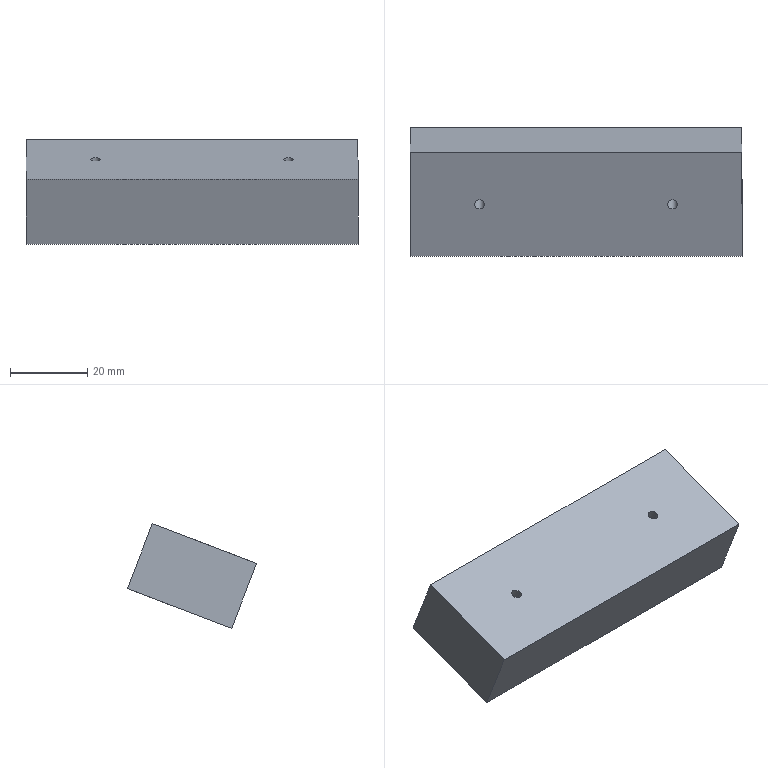Component | SolidWorks | CV-BA-74X27-1 | 1 solid | 19 faces | box 86 x 33.42 x 27.14 mm | volume 43255 mm3 | plane 11 | cylinder 4 | cone 4 | commonest cylinder face diameters 2.5 x4
build123d program:
from build123d import *

# Parameters (mm, degrees)
SKETCH1_W             = 86
SKETCH1_H             = 28.9
BOSS_EXTRUDE1_DEPTH   = 18
SKETCH2_W             = 57.364
SKETCH2_H             = 24.341
CUT_EXTRUDE1_DEPTH    = 1
M3_TAPPED_HOLE1_D     = 2.5
M3_TAPPED_HOLE1_DEPTH = 8.5
M3_TAPPED_HOLE1_TIP   = 0.7511


with BuildPart() as part:
    # Sketch1 → Boss-Extrude1 (new body)
    with BuildSketch(Plane.XY):
        Rectangle(SKETCH1_W, SKETCH1_H)
    extrude(amount=BOSS_EXTRUDE1_DEPTH)

    # Sketch2 → Cut-Extrude1 (cut)
    with BuildSketch(Plane.XY.offset(18)):
        Rectangle(SKETCH2_W, SKETCH2_H)
    extrude(amount=-CUT_EXTRUDE1_DEPTH, mode=Mode.SUBTRACT)

    # M3 Tapped Hole1
    with Locations(Plane(origin=(0, 0, 0), x_dir=(-1, 0, 0), z_dir=(0, 0, -1))):
        with Locations((-25, 0), (25, 0)):
            Hole(M3_TAPPED_HOLE1_D / 2, depth=M3_TAPPED_HOLE1_DEPTH)
            with Locations((0, 0, -(M3_TAPPED_HOLE1_DEPTH + M3_TAPPED_HOLE1_TIP / 2))):  # 118° drill point
                Cone(0, M3_TAPPED_HOLE1_D / 2, M3_TAPPED_HOLE1_TIP, mode=Mode.SUBTRACT)


solid = part.part

# Placed as in the assembly
solid = solid.moved(Location((-143.297, 122.354, 409.108), (-159.065, 0, 0)))
STEP:
#1=COLOUR_RGB('',0.7922,0.8196,0.9333);
#2=FILL_AREA_STYLE_COLOUR('',#1);
#3=FILL_AREA_STYLE('',(#2));
#4=SURFACE_STYLE_FILL_AREA(#3);
#5=SURFACE_SIDE_STYLE('',(#4));
#6=SURFACE_STYLE_USAGE(.BOTH.,#5);
#7=PRESENTATION_STYLE_ASSIGNMENT((#6));
#8=CARTESIAN_POINT('',(-4.608,4.937,15.794));
#9=VERTEX_POINT('',#8);
#10=CARTESIAN_POINT('',(-4.707,4.937,15.794));
#11=VERTEX_POINT('',#10);
#12=CARTESIAN_POINT('',(-4.657,4.937,15.794));
#13=DIRECTION('',(0.,-0.3573,0.934));
#14=DIRECTION('',(-1.,0.,0.));
#15=AXIS2_PLACEMENT_3D('',#12,#13,#14);
#16=CIRCLE('',#15,0.04921);
#17=EDGE_CURVE('',#9,#11,#16,.T.);
#18=ORIENTED_EDGE('',*,*,#17,.F.);
#19=CARTESIAN_POINT('',(-4.608,4.817,16.107));
#20=VERTEX_POINT('',#19);
#21=CARTESIAN_POINT('',(-4.608,4.817,16.107));
#22=DIRECTION('',(0.,-0.3573,0.934));
#23=VECTOR('',#22,39.37);
#24=LINE('',#21,#23);
#25=EDGE_CURVE('',#9,#20,#24,.T.);
#26=ORIENTED_EDGE('',*,*,#25,.T.);
#27=CARTESIAN_POINT('',(-4.707,4.817,16.107));
#28=VERTEX_POINT('',#27);
#29=CARTESIAN_POINT('',(-4.657,4.817,16.107));
#30=DIRECTION('',(0.,-0.3573,0.934));
#31=DIRECTION('',(-1.,0.,0.));
#32=AXIS2_PLACEMENT_3D('',#29,#30,#31);
#33=CIRCLE('',#32,0.04921);
#34=EDGE_CURVE('',#20,#28,#33,.T.);
#35=ORIENTED_EDGE('',*,*,#34,.T.);
#36=CARTESIAN_POINT('',(-4.707,4.817,16.107));
#37=DIRECTION('',(0.,-0.3573,0.934));
#38=VECTOR('',#37,39.37);
#39=LINE('',#36,#38);
#40=EDGE_CURVE('',#11,#28,#39,.T.);
#41=ORIENTED_EDGE('',*,*,#40,.F.);
#42=EDGE_LOOP('',(#18,#26,#35,#41));
#43=FACE_OUTER_BOUND('',#42,.T.);
#44=CARTESIAN_POINT('',(-4.657,4.817,16.107));
#45=DIRECTION('',(0.,-0.3573,0.934));
#46=DIRECTION('',(-1.,0.,0.));
#47=AXIS2_PLACEMENT_3D('',#44,#45,#46);
#48=CYLINDRICAL_SURFACE('',#47,0.04921);
#49=ADVANCED_FACE('',(#43),#48,.F.);
#50=CARTESIAN_POINT('',(-4.657,4.947,15.766));
#51=VERTEX_POINT('',#50);
#52=CARTESIAN_POINT('',(-4.707,4.937,15.794));
#53=DIRECTION('',(-0.8572,-0.184,0.481));
#54=VECTOR('',#53,39.37);
#55=LINE('',#52,#54);
#56=EDGE_CURVE('',#51,#11,#55,.T.);
#57=ORIENTED_EDGE('',*,*,#56,.F.);
#58=CARTESIAN_POINT('',(-4.608,4.937,15.794));
#59=DIRECTION('',(0.8572,-0.184,0.481));
#60=VECTOR('',#59,39.37);
#61=LINE('',#58,#60);
#62=EDGE_CURVE('',#51,#9,#61,.T.);
#63=ORIENTED_EDGE('',*,*,#62,.T.);
#64=ORIENTED_EDGE('',*,*,#17,.T.);
#65=EDGE_LOOP('',(#57,#63,#64));
#66=FACE_OUTER_BOUND('',#65,.T.);
#67=CARTESIAN_POINT('',(-4.657,4.937,15.794));
#68=DIRECTION('',(0.,-0.3573,0.934));
#69=DIRECTION('',(-1.,0.,0.));
#70=AXIS2_PLACEMENT_3D('',#67,#68,#69);
#71=CONICAL_SURFACE('',#70,0.04921,1.03);
#72=ADVANCED_FACE('',(#66),#71,.F.);
#73=CARTESIAN_POINT('',(-6.577,4.937,15.794));
#74=VERTEX_POINT('',#73);
#75=CARTESIAN_POINT('',(-6.675,4.937,15.794));
#76=VERTEX_POINT('',#75);
#77=CARTESIAN_POINT('',(-6.626,4.937,15.794));
#78=DIRECTION('',(0.,-0.3573,0.934));
#79=DIRECTION('',(-1.,0.,0.));
#80=AXIS2_PLACEMENT_3D('',#77,#78,#79);
#81=CIRCLE('',#80,0.04921);
#82=EDGE_CURVE('',#74,#76,#81,.T.);
#83=ORIENTED_EDGE('',*,*,#82,.F.);
#84=CARTESIAN_POINT('',(-6.577,4.817,16.107));
#85=VERTEX_POINT('',#84);
#86=CARTESIAN_POINT('',(-6.577,4.817,16.107));
#87=DIRECTION('',(0.,-0.3573,0.934));
#88=VECTOR('',#87,39.37);
#89=LINE('',#86,#88);
#90=EDGE_CURVE('',#74,#85,#89,.T.);
#91=ORIENTED_EDGE('',*,*,#90,.T.);
#92=CARTESIAN_POINT('',(-6.675,4.817,16.107));
#93=VERTEX_POINT('',#92);
#94=CARTESIAN_POINT('',(-6.626,4.817,16.107));
#95=DIRECTION('',(0.,-0.3573,0.934));
#96=DIRECTION('',(-1.,0.,0.));
#97=AXIS2_PLACEMENT_3D('',#94,#95,#96);
#98=CIRCLE('',#97,0.04921);
#99=EDGE_CURVE('',#85,#93,#98,.T.);
#100=ORIENTED_EDGE('',*,*,#99,.T.);
#101=CARTESIAN_POINT('',(-6.675,4.817,16.107));
#102=DIRECTION('',(0.,-0.3573,0.934));
#103=VECTOR('',#102,39.37);
#104=LINE('',#101,#103);
#105=EDGE_CURVE('',#76,#93,#104,.T.);
#106=ORIENTED_EDGE('',*,*,#105,.F.);
#107=EDGE_LOOP('',(#83,#91,#100,#106));
#108=FACE_OUTER_BOUND('',#107,.T.);
#109=CARTESIAN_POINT('',(-6.626,4.817,16.107));
#110=DIRECTION('',(0.,-0.3573,0.934));
#111=DIRECTION('',(-1.,0.,0.));
#112=AXIS2_PLACEMENT_3D('',#109,#110,#111);
#113=CYLINDRICAL_SURFACE('',#112,0.04921);
#114=ADVANCED_FACE('',(#108),#113,.F.);
#115=CARTESIAN_POINT('',(-6.626,4.947,15.766));
#116=VERTEX_POINT('',#115);
#117=CARTESIAN_POINT('',(-6.675,4.937,15.794));
#118=DIRECTION('',(-0.8572,-0.184,0.481));
#119=VECTOR('',#118,39.37);
#120=LINE('',#117,#119);
#121=EDGE_CURVE('',#116,#76,#120,.T.);
#122=ORIENTED_EDGE('',*,*,#121,.F.);
#123=CARTESIAN_POINT('',(-6.577,4.937,15.794));
#124=DIRECTION('',(0.8572,-0.184,0.481));
#125=VECTOR('',#124,39.37);
#126=LINE('',#123,#125);
#127=EDGE_CURVE('',#116,#74,#126,.T.);
#128=ORIENTED_EDGE('',*,*,#127,.T.);
#129=ORIENTED_EDGE('',*,*,#82,.T.);
#130=EDGE_LOOP('',(#122,#128,#129));
#131=FACE_OUTER_BOUND('',#130,.T.);
#132=CARTESIAN_POINT('',(-6.626,4.937,15.794));
#133=DIRECTION('',(0.,-0.3573,0.934));
#134=DIRECTION('',(-1.,0.,0.));
#135=AXIS2_PLACEMENT_3D('',#132,#133,#134);
#136=CONICAL_SURFACE('',#135,0.04921,1.03);
#137=ADVANCED_FACE('',(#131),#136,.F.);
#138=CARTESIAN_POINT('',(-3.949,5.348,16.31));
#139=VERTEX_POINT('',#138);
#140=CARTESIAN_POINT('',(-3.949,4.286,15.903));
#141=VERTEX_POINT('',#140);
#142=CARTESIAN_POINT('',(-3.949,4.286,15.903));
#143=DIRECTION('',(0.,-0.934,-0.3573));
#144=VECTOR('',#143,39.37);
#145=LINE('',#142,#144);
#146=EDGE_CURVE('',#139,#141,#145,.T.);
#147=ORIENTED_EDGE('',*,*,#146,.T.);
#148=CARTESIAN_POINT('',(-3.949,4.539,15.241));
#149=VERTEX_POINT('',#148);
#150=CARTESIAN_POINT('',(-3.949,4.539,15.241));
#151=DIRECTION('',(0.,-0.3573,0.934));
#152=VECTOR('',#151,39.37);
#153=LINE('',#150,#152);
#154=EDGE_CURVE('',#149,#141,#153,.T.);
#155=ORIENTED_EDGE('',*,*,#154,.F.);
#156=CARTESIAN_POINT('',(-3.949,5.602,15.648));
#157=VERTEX_POINT('',#156);
#158=CARTESIAN_POINT('',(-3.949,4.539,15.241));
#159=DIRECTION('',(0.,-0.934,-0.3573));
#160=VECTOR('',#159,39.37);
#161=LINE('',#158,#160);
#162=EDGE_CURVE('',#157,#149,#161,.T.);
#163=ORIENTED_EDGE('',*,*,#162,.F.);
#164=CARTESIAN_POINT('',(-3.949,5.602,15.648));
#165=DIRECTION('',(0.,-0.3573,0.934));
#166=VECTOR('',#165,39.37);
#167=LINE('',#164,#166);
#168=EDGE_CURVE('',#157,#139,#167,.T.);
#169=ORIENTED_EDGE('',*,*,#168,.T.);
#170=EDGE_LOOP('',(#147,#155,#163,#169));
#171=FACE_OUTER_BOUND('',#170,.T.);
#172=CARTESIAN_POINT('',(-3.949,4.539,15.241));
#173=DIRECTION('',(-1.,-0.,0.));
#174=DIRECTION('',(-0.,0.3573,-0.934));
#175=AXIS2_PLACEMENT_3D('',#172,#173,#174);
#176=PLANE('',#175);
#177=ADVANCED_FACE('',(#171),#176,.F.);
#178=CARTESIAN_POINT('',(-7.335,4.286,15.903));
#179=VERTEX_POINT('',#178);
#180=CARTESIAN_POINT('',(-7.335,4.286,15.903));
#181=DIRECTION('',(-1.,-0.,0.));
#182=VECTOR('',#181,39.37);
#183=LINE('',#180,#182);
#184=EDGE_CURVE('',#141,#179,#183,.T.);
#185=ORIENTED_EDGE('',*,*,#184,.T.);
#186=CARTESIAN_POINT('',(-7.335,4.539,15.241));
#187=VERTEX_POINT('',#186);
#188=CARTESIAN_POINT('',(-7.335,4.539,15.241));
#189=DIRECTION('',(0.,-0.3573,0.934));
#190=VECTOR('',#189,39.37);
#191=LINE('',#188,#190);
#192=EDGE_CURVE('',#187,#179,#191,.T.);
#193=ORIENTED_EDGE('',*,*,#192,.F.);
#194=CARTESIAN_POINT('',(-7.335,4.539,15.241));
#195=DIRECTION('',(-1.,-0.,0.));
#196=VECTOR('',#195,39.37);
#197=LINE('',#194,#196);
#198=EDGE_CURVE('',#149,#187,#197,.T.);
#199=ORIENTED_EDGE('',*,*,#198,.F.);
#200=ORIENTED_EDGE('',*,*,#154,.T.);
#201=EDGE_LOOP('',(#185,#193,#199,#200));
#202=FACE_OUTER_BOUND('',#201,.T.);
#203=CARTESIAN_POINT('',(-7.335,4.539,15.241));
#204=DIRECTION('',(-0.,0.934,0.3573));
#205=DIRECTION('',(0.,-0.3573,0.934));
#206=AXIS2_PLACEMENT_3D('',#203,#204,#205);
#207=PLANE('',#206);
#208=ADVANCED_FACE('',(#202),#207,.F.);
#209=CARTESIAN_POINT('',(-7.335,5.348,16.31));
#210=VERTEX_POINT('',#209);
#211=CARTESIAN_POINT('',(-7.335,4.286,15.903));
#212=DIRECTION('',(0.,0.934,0.3573));
#213=VECTOR('',#212,39.37);
#214=LINE('',#211,#213);
#215=EDGE_CURVE('',#179,#210,#214,.T.);
#216=ORIENTED_EDGE('',*,*,#215,.T.);
#217=CARTESIAN_POINT('',(-7.335,5.602,15.648));
#218=VERTEX_POINT('',#217);
#219=CARTESIAN_POINT('',(-7.335,5.602,15.648));
#220=DIRECTION('',(0.,-0.3573,0.934));
#221=VECTOR('',#220,39.37);
#222=LINE('',#219,#221);
#223=EDGE_CURVE('',#218,#210,#222,.T.);
#224=ORIENTED_EDGE('',*,*,#223,.F.);
#225=CARTESIAN_POINT('',(-7.335,4.539,15.241));
#226=DIRECTION('',(0.,0.934,0.3573));
#227=VECTOR('',#226,39.37);
#228=LINE('',#225,#227);
#229=EDGE_CURVE('',#187,#218,#228,.T.);
#230=ORIENTED_EDGE('',*,*,#229,.F.);
#231=ORIENTED_EDGE('',*,*,#192,.T.);
#232=EDGE_LOOP('',(#216,#224,#230,#231));
#233=FACE_OUTER_BOUND('',#232,.T.);
#234=CARTESIAN_POINT('',(-7.335,4.539,15.241));
#235=DIRECTION('',(1.,-0.,-0.));
#236=DIRECTION('',(-0.,-0.934,-0.3573));
#237=AXIS2_PLACEMENT_3D('',#234,#235,#236);
#238=PLANE('',#237);
#239=ADVANCED_FACE('',(#233),#238,.F.);
#240=CARTESIAN_POINT('',(-7.335,5.348,16.31));
#241=DIRECTION('',(1.,0.,-0.));
#242=VECTOR('',#241,39.37);
#243=LINE('',#240,#242);
#244=EDGE_CURVE('',#210,#139,#243,.T.);
#245=ORIENTED_EDGE('',*,*,#244,.T.);
#246=ORIENTED_EDGE('',*,*,#168,.F.);
#247=CARTESIAN_POINT('',(-7.335,5.602,15.648));
#248=DIRECTION('',(1.,0.,-0.));
#249=VECTOR('',#248,39.37);
#250=LINE('',#247,#249);
#251=EDGE_CURVE('',#218,#157,#250,.T.);
#252=ORIENTED_EDGE('',*,*,#251,.F.);
#253=ORIENTED_EDGE('',*,*,#223,.T.);
#254=EDGE_LOOP('',(#245,#246,#252,#253));
#255=FACE_OUTER_BOUND('',#254,.T.);
#256=CARTESIAN_POINT('',(-7.335,5.602,15.648));
#257=DIRECTION('',(0.,-0.934,-0.3573));
#258=DIRECTION('',(-0.,0.3573,-0.934));
#259=AXIS2_PLACEMENT_3D('',#256,#257,#258);
#260=PLANE('',#259);
#261=ADVANCED_FACE('',(#255),#260,.F.);
#262=CARTESIAN_POINT('',(-4.512,5.518,15.616));
#263=VERTEX_POINT('',#262);
#264=CARTESIAN_POINT('',(-4.512,4.623,15.274));
#265=VERTEX_POINT('',#264);
#266=CARTESIAN_POINT('',(-4.512,4.623,15.274));
#267=DIRECTION('',(0.,-0.934,-0.3573));
#268=VECTOR('',#267,39.37);
#269=LINE('',#266,#268);
#270=EDGE_CURVE('',#263,#265,#269,.T.);
#271=ORIENTED_EDGE('',*,*,#270,.F.);
#272=CARTESIAN_POINT('',(-6.771,5.518,15.616));
#273=VERTEX_POINT('',#272);
#274=CARTESIAN_POINT('',(-6.771,5.518,15.616));
#275=DIRECTION('',(1.,0.,0.));
#276=VECTOR('',#275,39.37);
#277=LINE('',#274,#276);
#278=EDGE_CURVE('',#273,#263,#277,.T.);
#279=ORIENTED_EDGE('',*,*,#278,.F.);
#280=CARTESIAN_POINT('',(-6.771,4.623,15.274));
#281=VERTEX_POINT('',#280);
#282=CARTESIAN_POINT('',(-6.771,4.623,15.274));
#283=DIRECTION('',(0.,0.934,0.3573));
#284=VECTOR('',#283,39.37);
#285=LINE('',#282,#284);
#286=EDGE_CURVE('',#281,#273,#285,.T.);
#287=ORIENTED_EDGE('',*,*,#286,.F.);
#288=CARTESIAN_POINT('',(-6.771,4.623,15.274));
#289=DIRECTION('',(-1.,-0.,0.));
#290=VECTOR('',#289,39.37);
#291=LINE('',#288,#290);
#292=EDGE_CURVE('',#265,#281,#291,.T.);
#293=ORIENTED_EDGE('',*,*,#292,.F.);
#294=EDGE_LOOP('',(#271,#279,#287,#293));
#295=FACE_BOUND('',#294,.T.);
#296=ORIENTED_EDGE('',*,*,#162,.T.);
#297=ORIENTED_EDGE('',*,*,#198,.T.);
#298=ORIENTED_EDGE('',*,*,#229,.T.);
#299=ORIENTED_EDGE('',*,*,#251,.T.);
#300=EDGE_LOOP('',(#296,#297,#298,#299));
#301=FACE_OUTER_BOUND('',#300,.T.);
#302=CARTESIAN_POINT('',(-5.642,5.07,15.445));
#303=DIRECTION('',(-0.,0.3573,-0.934));
#304=DIRECTION('',(1.,0.,-0.));
#305=AXIS2_PLACEMENT_3D('',#302,#303,#304);
#306=PLANE('',#305);
#307=ADVANCED_FACE('',(#295,#301),#306,.T.);
#308=CARTESIAN_POINT('',(-4.657,4.817,16.107));
#309=DIRECTION('',(0.,-0.3573,0.934));
#310=DIRECTION('',(-1.,0.,0.));
#311=AXIS2_PLACEMENT_3D('',#308,#309,#310);
#312=CIRCLE('',#311,0.04921);
#313=EDGE_CURVE('',#28,#20,#312,.T.);
#314=ORIENTED_EDGE('',*,*,#313,.F.);
#315=ORIENTED_EDGE('',*,*,#34,.F.);
#316=EDGE_LOOP('',(#314,#315));
#317=FACE_BOUND('',#316,.T.);
#318=CARTESIAN_POINT('',(-6.626,4.817,16.107));
#319=DIRECTION('',(0.,-0.3573,0.934));
#320=DIRECTION('',(-1.,0.,0.));
#321=AXIS2_PLACEMENT_3D('',#318,#319,#320);
#322=CIRCLE('',#321,0.04921);
#323=EDGE_CURVE('',#93,#85,#322,.T.);
#324=ORIENTED_EDGE('',*,*,#323,.F.);
#325=ORIENTED_EDGE('',*,*,#99,.F.);
#326=EDGE_LOOP('',(#324,#325));
#327=FACE_BOUND('',#326,.T.);
#328=ORIENTED_EDGE('',*,*,#146,.F.);
#329=ORIENTED_EDGE('',*,*,#244,.F.);
#330=ORIENTED_EDGE('',*,*,#215,.F.);
#331=ORIENTED_EDGE('',*,*,#184,.F.);
#332=EDGE_LOOP('',(#328,#329,#330,#331));
#333=FACE_OUTER_BOUND('',#332,.T.);
#334=CARTESIAN_POINT('',(-5.642,4.817,16.107));
#335=DIRECTION('',(-0.,0.3573,-0.934));
#336=DIRECTION('',(1.,0.,-0.));
#337=AXIS2_PLACEMENT_3D('',#334,#335,#336);
#338=PLANE('',#337);
#339=ADVANCED_FACE('',(#317,#327,#333),#338,.F.);
#340=ORIENTED_EDGE('',*,*,#270,.T.);
#341=CARTESIAN_POINT('',(-4.512,4.609,15.31));
#342=VERTEX_POINT('',#341);
#343=CARTESIAN_POINT('',(-4.512,4.609,15.31));
#344=DIRECTION('',(-0.,0.3573,-0.934));
#345=VECTOR('',#344,39.37);
#346=LINE('',#343,#345);
#347=EDGE_CURVE('',#342,#265,#346,.T.);
#348=ORIENTED_EDGE('',*,*,#347,.F.);
#349=CARTESIAN_POINT('',(-4.512,5.504,15.653));
#350=VERTEX_POINT('',#349);
#351=CARTESIAN_POINT('',(-4.512,4.609,15.31));
#352=DIRECTION('',(0.,-0.934,-0.3573));
#353=VECTOR('',#352,39.37);
#354=LINE('',#351,#353);
#355=EDGE_CURVE('',#350,#342,#354,.T.);
#356=ORIENTED_EDGE('',*,*,#355,.F.);
#357=CARTESIAN_POINT('',(-4.512,5.504,15.653));
#358=DIRECTION('',(-0.,0.3573,-0.934));
#359=VECTOR('',#358,39.37);
#360=LINE('',#357,#359);
#361=EDGE_CURVE('',#350,#263,#360,.T.);
#362=ORIENTED_EDGE('',*,*,#361,.T.);
#363=EDGE_LOOP('',(#340,#348,#356,#362));
#364=FACE_OUTER_BOUND('',#363,.T.);
#365=CARTESIAN_POINT('',(-4.512,4.609,15.31));
#366=DIRECTION('',(1.,0.,-0.));
#367=DIRECTION('',(0.,-0.3573,0.934));
#368=AXIS2_PLACEMENT_3D('',#365,#366,#367);
#369=PLANE('',#368);
#370=ADVANCED_FACE('',(#364),#369,.F.);
#371=ORIENTED_EDGE('',*,*,#278,.T.);
#372=ORIENTED_EDGE('',*,*,#361,.F.);
#373=CARTESIAN_POINT('',(-6.771,5.504,15.653));
#374=VERTEX_POINT('',#373);
#375=CARTESIAN_POINT('',(-6.771,5.504,15.653));
#376=DIRECTION('',(1.,0.,0.));
#377=VECTOR('',#376,39.37);
#378=LINE('',#375,#377);
#379=EDGE_CURVE('',#374,#350,#378,.T.);
#380=ORIENTED_EDGE('',*,*,#379,.F.);
#381=CARTESIAN_POINT('',(-6.771,5.504,15.653));
#382=DIRECTION('',(-0.,0.3573,-0.934));
#383=VECTOR('',#382,39.37);
#384=LINE('',#381,#383);
#385=EDGE_CURVE('',#374,#273,#384,.T.);
#386=ORIENTED_EDGE('',*,*,#385,.T.);
#387=EDGE_LOOP('',(#371,#372,#380,#386));
#388=FACE_OUTER_BOUND('',#387,.T.);
#389=CARTESIAN_POINT('',(-6.771,5.504,15.653));
#390=DIRECTION('',(-0.,0.934,0.3573));
#391=DIRECTION('',(1.,0.,0.));
#392=AXIS2_PLACEMENT_3D('',#389,#390,#391);
#393=PLANE('',#392);
#394=ADVANCED_FACE('',(#388),#393,.F.);
#395=ORIENTED_EDGE('',*,*,#286,.T.);
#396=ORIENTED_EDGE('',*,*,#385,.F.);
#397=CARTESIAN_POINT('',(-6.771,4.609,15.31));
#398=VERTEX_POINT('',#397);
#399=CARTESIAN_POINT('',(-6.771,4.609,15.31));
#400=DIRECTION('',(0.,0.934,0.3573));
#401=VECTOR('',#400,39.37);
#402=LINE('',#399,#401);
#403=EDGE_CURVE('',#398,#374,#402,.T.);
#404=ORIENTED_EDGE('',*,*,#403,.F.);
#405=CARTESIAN_POINT('',(-6.771,4.609,15.31));
#406=DIRECTION('',(-0.,0.3573,-0.934));
#407=VECTOR('',#406,39.37);
#408=LINE('',#405,#407);
#409=EDGE_CURVE('',#398,#281,#408,.T.);
#410=ORIENTED_EDGE('',*,*,#409,.T.);
#411=EDGE_LOOP('',(#395,#396,#404,#410));
#412=FACE_OUTER_BOUND('',#411,.T.);
#413=CARTESIAN_POINT('',(-6.771,4.609,15.31));
#414=DIRECTION('',(-1.,-0.,0.));
#415=DIRECTION('',(0.,0.934,0.3573));
#416=AXIS2_PLACEMENT_3D('',#413,#414,#415);
#417=PLANE('',#416);
#418=ADVANCED_FACE('',(#412),#417,.F.);
#419=ORIENTED_EDGE('',*,*,#292,.T.);
#420=ORIENTED_EDGE('',*,*,#409,.F.);
#421=CARTESIAN_POINT('',(-6.771,4.609,15.31));
#422=DIRECTION('',(-1.,-0.,0.));
#423=VECTOR('',#422,39.37);
#424=LINE('',#421,#423);
#425=EDGE_CURVE('',#342,#398,#424,.T.);
#426=ORIENTED_EDGE('',*,*,#425,.F.);
#427=ORIENTED_EDGE('',*,*,#347,.T.);
#428=EDGE_LOOP('',(#419,#420,#426,#427));
#429=FACE_OUTER_BOUND('',#428,.T.);
#430=CARTESIAN_POINT('',(-6.771,4.609,15.31));
#431=DIRECTION('',(0.,-0.934,-0.3573));
#432=DIRECTION('',(-0.,0.3573,-0.934));
#433=AXIS2_PLACEMENT_3D('',#430,#431,#432);
#434=PLANE('',#433);
#435=ADVANCED_FACE('',(#429),#434,.F.);
#436=ORIENTED_EDGE('',*,*,#355,.T.);
#437=ORIENTED_EDGE('',*,*,#425,.T.);
#438=ORIENTED_EDGE('',*,*,#403,.T.);
#439=ORIENTED_EDGE('',*,*,#379,.T.);
#440=EDGE_LOOP('',(#436,#437,#438,#439));
#441=FACE_OUTER_BOUND('',#440,.T.);
#442=CARTESIAN_POINT('',(-5.642,5.056,15.482));
#443=DIRECTION('',(-0.,0.3573,-0.934));
#444=DIRECTION('',(1.,0.,-0.));
#445=AXIS2_PLACEMENT_3D('',#442,#443,#444);
#446=PLANE('',#445);
#447=ADVANCED_FACE('',(#441),#446,.T.);
#448=ORIENTED_EDGE('',*,*,#127,.F.);
#449=ORIENTED_EDGE('',*,*,#121,.T.);
#450=CARTESIAN_POINT('',(-6.626,4.937,15.794));
#451=DIRECTION('',(0.,-0.3573,0.934));
#452=DIRECTION('',(-1.,0.,0.));
#453=AXIS2_PLACEMENT_3D('',#450,#451,#452);
#454=CIRCLE('',#453,0.04921);
#455=EDGE_CURVE('',#76,#74,#454,.T.);
#456=ORIENTED_EDGE('',*,*,#455,.T.);
#457=EDGE_LOOP('',(#448,#449,#456));
#458=FACE_OUTER_BOUND('',#457,.T.);
#459=CARTESIAN_POINT('',(-6.626,4.937,15.794));
#460=DIRECTION('',(0.,-0.3573,0.934));
#461=DIRECTION('',(-1.,0.,0.));
#462=AXIS2_PLACEMENT_3D('',#459,#460,#461);
#463=CONICAL_SURFACE('',#462,0.04921,1.03);
#464=ADVANCED_FACE('',(#458),#463,.F.);
#465=ORIENTED_EDGE('',*,*,#90,.F.);
#466=ORIENTED_EDGE('',*,*,#455,.F.);
#467=ORIENTED_EDGE('',*,*,#105,.T.);
#468=ORIENTED_EDGE('',*,*,#323,.T.);
#469=EDGE_LOOP('',(#465,#466,#467,#468));
#470=FACE_OUTER_BOUND('',#469,.T.);
#471=CARTESIAN_POINT('',(-6.626,4.817,16.107));
#472=DIRECTION('',(0.,-0.3573,0.934));
#473=DIRECTION('',(-1.,0.,0.));
#474=AXIS2_PLACEMENT_3D('',#471,#472,#473);
#475=CYLINDRICAL_SURFACE('',#474,0.04921);
#476=ADVANCED_FACE('',(#470),#475,.F.);
#477=ORIENTED_EDGE('',*,*,#62,.F.);
#478=ORIENTED_EDGE('',*,*,#56,.T.);
#479=CARTESIAN_POINT('',(-4.657,4.937,15.794));
#480=DIRECTION('',(0.,-0.3573,0.934));
#481=DIRECTION('',(-1.,0.,0.));
#482=AXIS2_PLACEMENT_3D('',#479,#480,#481);
#483=CIRCLE('',#482,0.04921);
#484=EDGE_CURVE('',#11,#9,#483,.T.);
#485=ORIENTED_EDGE('',*,*,#484,.T.);
#486=EDGE_LOOP('',(#477,#478,#485));
#487=FACE_OUTER_BOUND('',#486,.T.);
#488=CARTESIAN_POINT('',(-4.657,4.937,15.794));
#489=DIRECTION('',(0.,-0.3573,0.934));
#490=DIRECTION('',(-1.,0.,0.));
#491=AXIS2_PLACEMENT_3D('',#488,#489,#490);
#492=CONICAL_SURFACE('',#491,0.04921,1.03);
#493=ADVANCED_FACE('',(#487),#492,.F.);
#494=ORIENTED_EDGE('',*,*,#25,.F.);
#495=ORIENTED_EDGE('',*,*,#484,.F.);
#496=ORIENTED_EDGE('',*,*,#40,.T.);
#497=ORIENTED_EDGE('',*,*,#313,.T.);
#498=EDGE_LOOP('',(#494,#495,#496,#497));
#499=FACE_OUTER_BOUND('',#498,.T.);
#500=CARTESIAN_POINT('',(-4.657,4.817,16.107));
#501=DIRECTION('',(0.,-0.3573,0.934));
#502=DIRECTION('',(-1.,0.,0.));
#503=AXIS2_PLACEMENT_3D('',#500,#501,#502);
#504=CYLINDRICAL_SURFACE('',#503,0.04921);
#505=ADVANCED_FACE('',(#499),#504,.F.);
#506=CLOSED_SHELL('',(#49,#72,#114,#137,#177,#208,#239,#261,#307,#339,#370,#394,#418,#435,#447,#464,#476,#493,#505));
#507=MANIFOLD_SOLID_BREP('',#506);
#508=STYLED_ITEM('',(#7),#507);
#509=(LENGTH_UNIT()NAMED_UNIT(*)SI_UNIT($,.METRE.));
#510=LENGTH_MEASURE_WITH_UNIT(LENGTH_MEASURE(0.0254),#509);
#511=DIMENSIONAL_EXPONENTS(1.,0.,0.,0.,0.,0.,0.);
#512=(CONVERSION_BASED_UNIT('',#510)LENGTH_UNIT()NAMED_UNIT(#511));
#513=UNCERTAINTY_MEASURE_WITH_UNIT(LENGTH_MEASURE(0.00001),#512,'','');
#514=(NAMED_UNIT(*)PLANE_ANGLE_UNIT()SI_UNIT($,.RADIAN.));
#515=(NAMED_UNIT(*)SI_UNIT($,.STERADIAN.)SOLID_ANGLE_UNIT());
#516=(GEOMETRIC_REPRESENTATION_CONTEXT(3)GLOBAL_UNCERTAINTY_ASSIGNED_CONTEXT((#513))GLOBAL_UNIT_ASSIGNED_CONTEXT((#512,#514,#515))REPRESENTATION_CONTEXT('',''));
#517=MECHANICAL_DESIGN_GEOMETRIC_PRESENTATION_REPRESENTATION('',(#508),#516);
#518=PRESENTATION_LAYER_ASSIGNMENT('','',(#508));
#519=CARTESIAN_POINT('',(0.,0.,0.));
#520=DIRECTION('',(0.,0.,1.));
#521=DIRECTION('',(1.,0.,0.));
#522=AXIS2_PLACEMENT_3D('',#519,#520,#521);
#523=(LENGTH_UNIT()NAMED_UNIT(*)SI_UNIT($,.METRE.));
#524=LENGTH_MEASURE_WITH_UNIT(LENGTH_MEASURE(0.0254),#523);
#525=DIMENSIONAL_EXPONENTS(1.,0.,0.,0.,0.,0.,0.);
#526=(CONVERSION_BASED_UNIT('',#524)LENGTH_UNIT()NAMED_UNIT(#525));
#527=UNCERTAINTY_MEASURE_WITH_UNIT(LENGTH_MEASURE(0.00001),#526,'','');
#528=(NAMED_UNIT(*)PLANE_ANGLE_UNIT()SI_UNIT($,.RADIAN.));
#529=(NAMED_UNIT(*)SI_UNIT($,.STERADIAN.)SOLID_ANGLE_UNIT());
#530=(GEOMETRIC_REPRESENTATION_CONTEXT(3)GLOBAL_UNCERTAINTY_ASSIGNED_CONTEXT((#527))GLOBAL_UNIT_ASSIGNED_CONTEXT((#526,#528,#529))REPRESENTATION_CONTEXT('',''));
#531=ADVANCED_BREP_SHAPE_REPRESENTATION('',(#507,#522),#530);